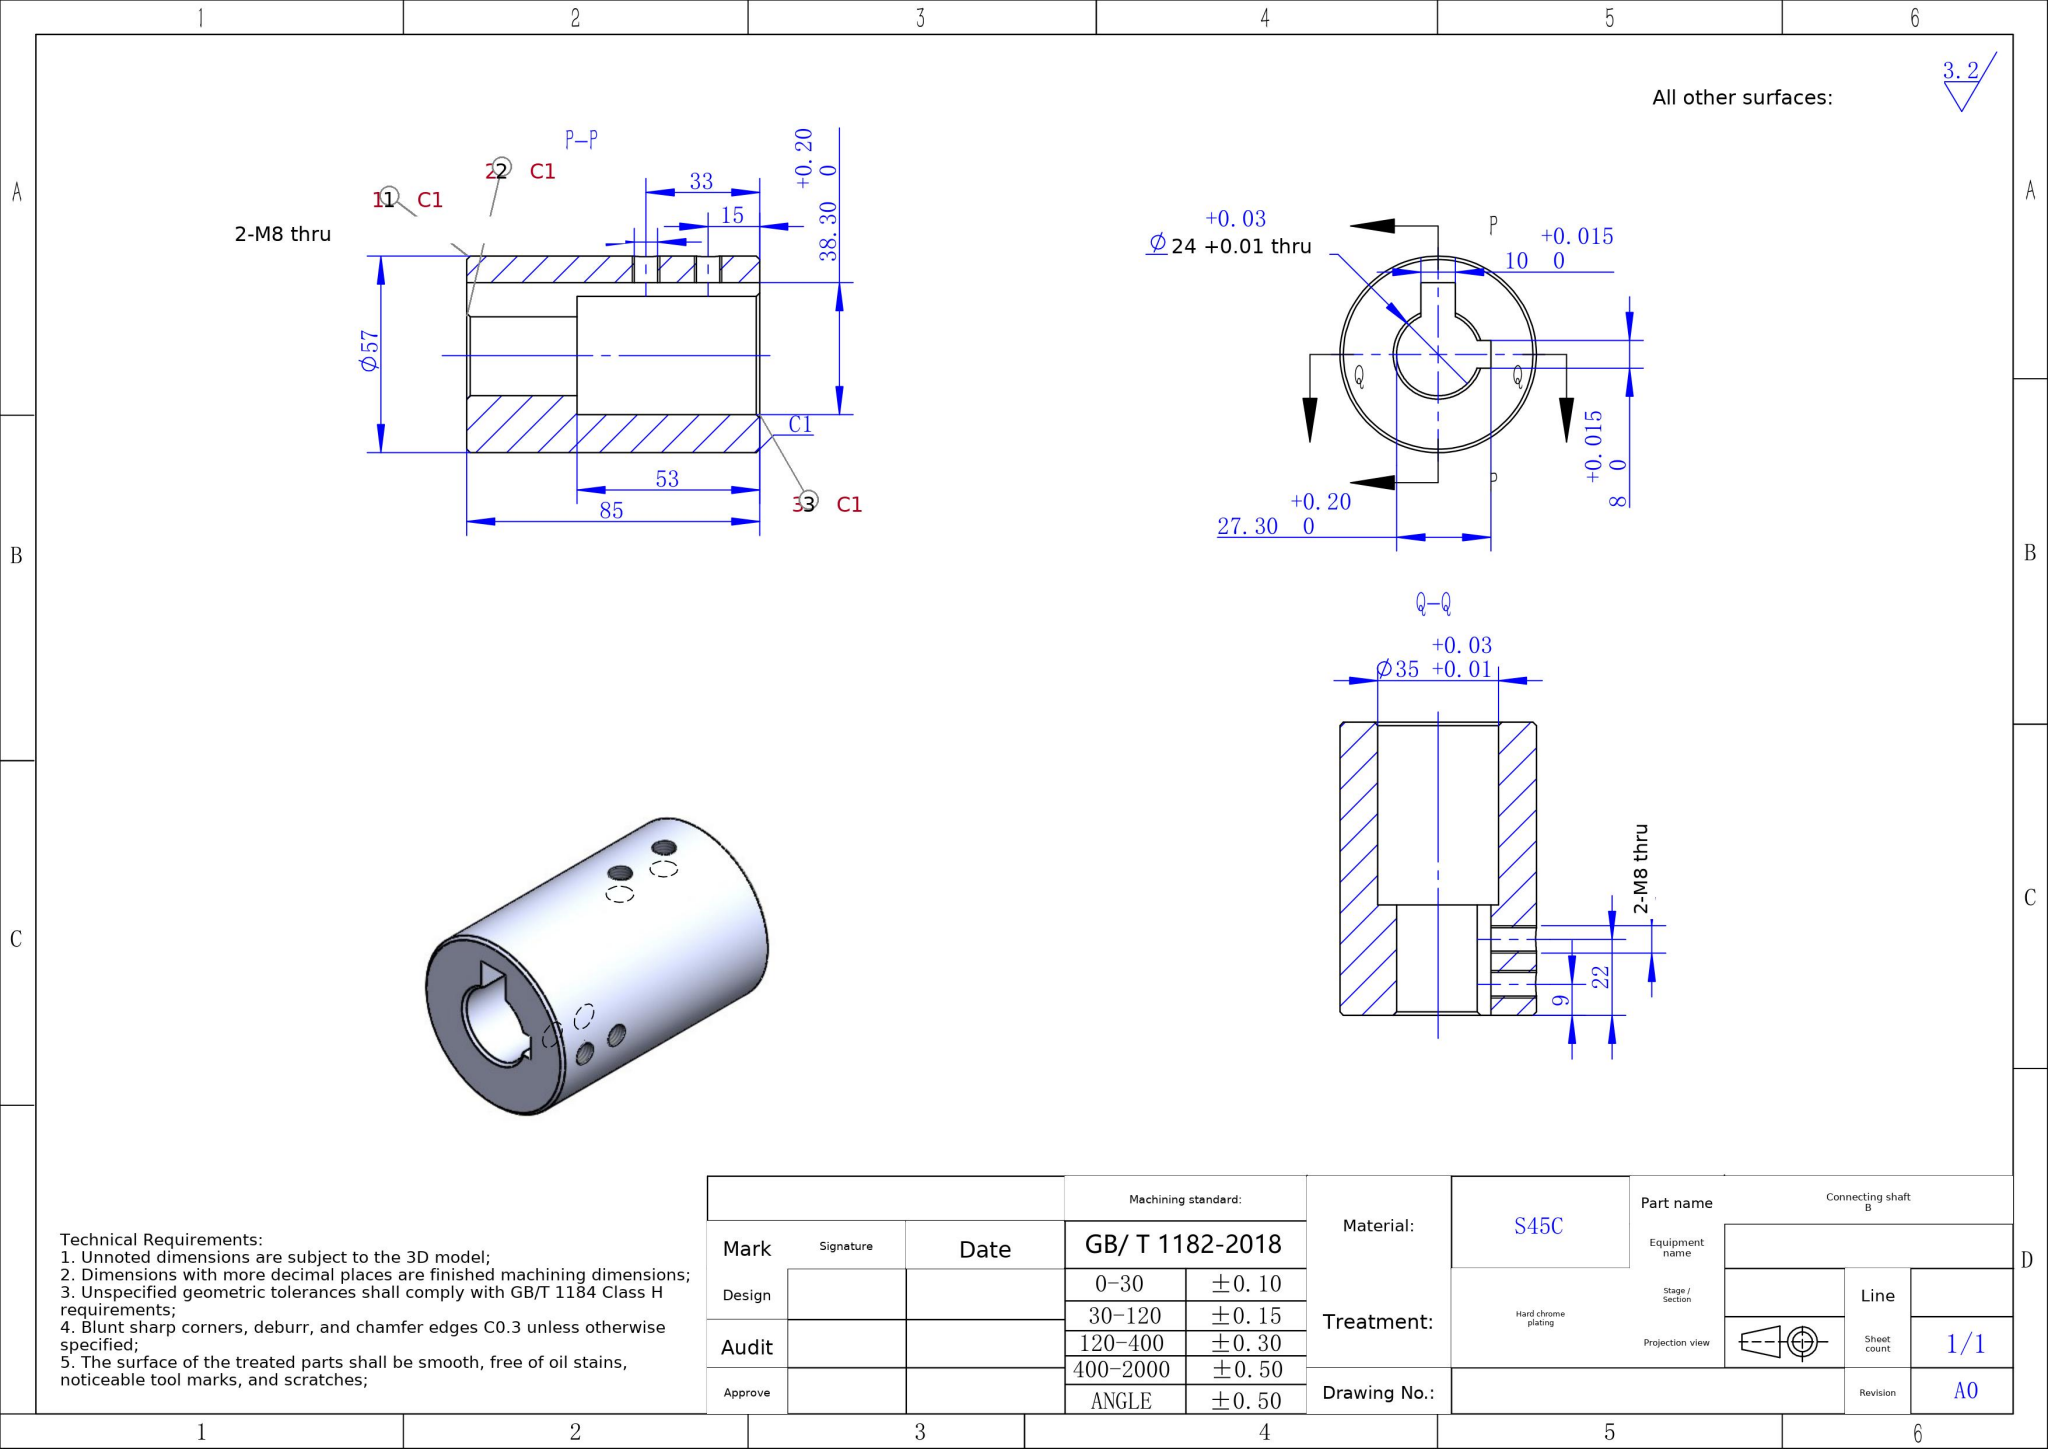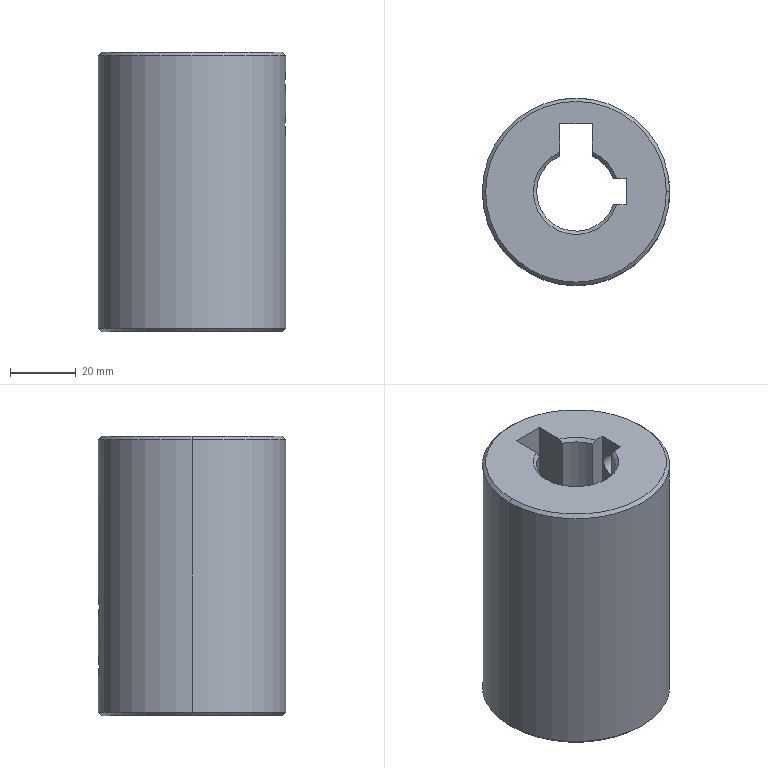Part | SolidWorks | mm | material S45C | 1 solid | 34 faces | box 57 x 57 x 85 mm | volume 143953 mm3 | cylinder 16 | cone 9 | plane 9 | commonest cylinder face diameters 6.8 x8 35 x3 24 x3 57 x2
build123d program:
from build123d import *

# Parameters (mm, degrees)
SKETCH1_R             = 28.5
BOSS_EXTRUDE1_DEPTH   = 85
SKETCH2_R             = 17.5
CUT_EXTRUDE1_DEPTH    = 53
SKETCH3_R             = 12
CUT_EXTRUDE2_DEPTH    = 67.585
CHAMFER1_SIZE         = 1
SKETCH4_W             = 10
SKETCH4_H             = 20
CUT_EXTRUDE3_DEPTH    = 95.072
SKETCH5_W             = 23.177
SKETCH5_H             = 8
CUT_EXTRUDE4_DEPTH    = 53
M8_TAPPED_HOLE1_D     = 6.8
M8_TAPPED_HOLE1_DEPTH = 22.25
M8_TAPPED_HOLE1_TIP   = 2.043
M8_TAPPED_HOLE2_D     = 6.8
M8_TAPPED_HOLE2_DEPTH = 22.25
M8_TAPPED_HOLE2_TIP   = 2.043
CHAMFER2_SIZE         = 1
CHAMFER3_SIZE         = 1


with BuildPart() as part:
    # Sketch1 → Boss-Extrude1 (new body)
    with BuildSketch(Plane.XY):
        Circle(SKETCH1_R)
    extrude(amount=BOSS_EXTRUDE1_DEPTH)

    # Sketch2 → Cut-Extrude1 (cut)
    with BuildSketch(Plane(origin=(0, 0, 0), x_dir=(-1, 0, 0), z_dir=(0, 0, -1))):
        Circle(SKETCH2_R)
    extrude(amount=-CUT_EXTRUDE1_DEPTH, mode=Mode.SUBTRACT)

    # Sketch3 → Cut-Extrude2 (cut, through all)
    with BuildSketch(Plane(origin=(0, 0, 53), x_dir=(-1, 0, 0), z_dir=(0, 0, -1))):
        Circle(SKETCH3_R)
    extrude(amount=-CUT_EXTRUDE2_DEPTH, mode=Mode.SUBTRACT)

    # Chamfer1
    chamfer1_edges = [part.edges().sort_by_distance(p)[0] for p in [
        (-28.5, 0, 0),
        (-28.5, 0, 85),
    ]]
    chamfer(chamfer1_edges, length=CHAMFER1_SIZE)

    # Sketch4 → Cut-Extrude3 (cut, through all)
    with BuildSketch(Plane(origin=(0, 0, 0), x_dir=(-1, 0, 0), z_dir=(0, 0, -1))):
        with Locations((0, 10.8)):
            Rectangle(SKETCH4_W, SKETCH4_H)
    extrude(amount=-CUT_EXTRUDE3_DEPTH, mode=Mode.SUBTRACT)

    # Sketch5 → Cut-Extrude4 (cut)
    with BuildSketch(Plane.XY.offset(85)):
        with Locations((3.712, 0)):
            Rectangle(SKETCH5_W, SKETCH5_H)
    extrude(amount=-CUT_EXTRUDE4_DEPTH, mode=Mode.SUBTRACT)

    # M8 Tapped Hole1
    with Locations(Plane(origin=(0, 28.5, 0), x_dir=(1, 0, 0), z_dir=(0, 1, 0))):
        with Locations((0, -15), (0, -33)):
            Hole(M8_TAPPED_HOLE1_D / 2, depth=M8_TAPPED_HOLE1_DEPTH)
            with Locations((0, 0, -(M8_TAPPED_HOLE1_DEPTH + M8_TAPPED_HOLE1_TIP / 2))):  # 118° drill point
                Cone(0, M8_TAPPED_HOLE1_D / 2, M8_TAPPED_HOLE1_TIP, mode=Mode.SUBTRACT)

    # M8 Tapped Hole2
    with Locations(Plane(origin=(28.5, 0, 85), x_dir=(0, 0, -1), z_dir=(1, 0, 0))):
        with Locations((9, 0), (22, 0)):
            Hole(M8_TAPPED_HOLE2_D / 2, depth=M8_TAPPED_HOLE2_DEPTH)
            with Locations((0, 0, -(M8_TAPPED_HOLE2_DEPTH + M8_TAPPED_HOLE2_TIP / 2))):  # 118° drill point
                Cone(0, M8_TAPPED_HOLE2_D / 2, M8_TAPPED_HOLE2_TIP, mode=Mode.SUBTRACT)

    # Chamfer2
    chamfer2_edges = [part.edges().sort_by_distance(p)[0] for p in [
        (8.858, 8.095, 85),
        (-8.095, -8.858, 85),
    ]]
    chamfer(chamfer2_edges, length=CHAMFER2_SIZE)

    # Chamfer3
    chamfer3_edges = [part.edges().sort_by_distance(p)[0] for p in [
        (0, -17.5, 0),
    ]]
    chamfer(chamfer3_edges, length=CHAMFER3_SIZE)


solid = part.part